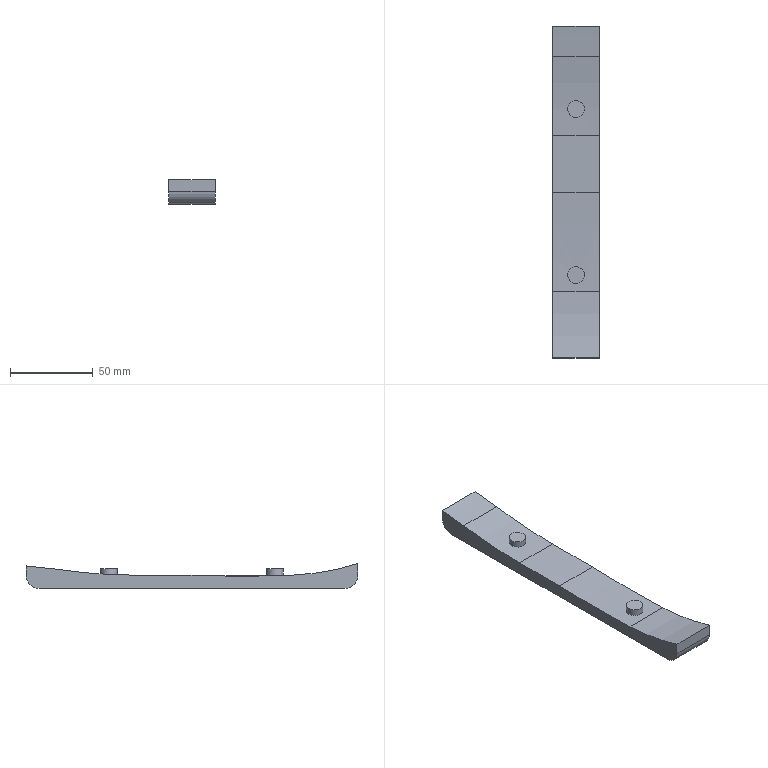Component | NX | CLOCKBASE1 | 1 solid | 16 faces | volume 50854 mm3 | plane 8 | cylinder 8 | commonest cylinder face diameters 16 x2 10 x2 300.087 x1 1600 x1 629.286 x1 1600.8 x1